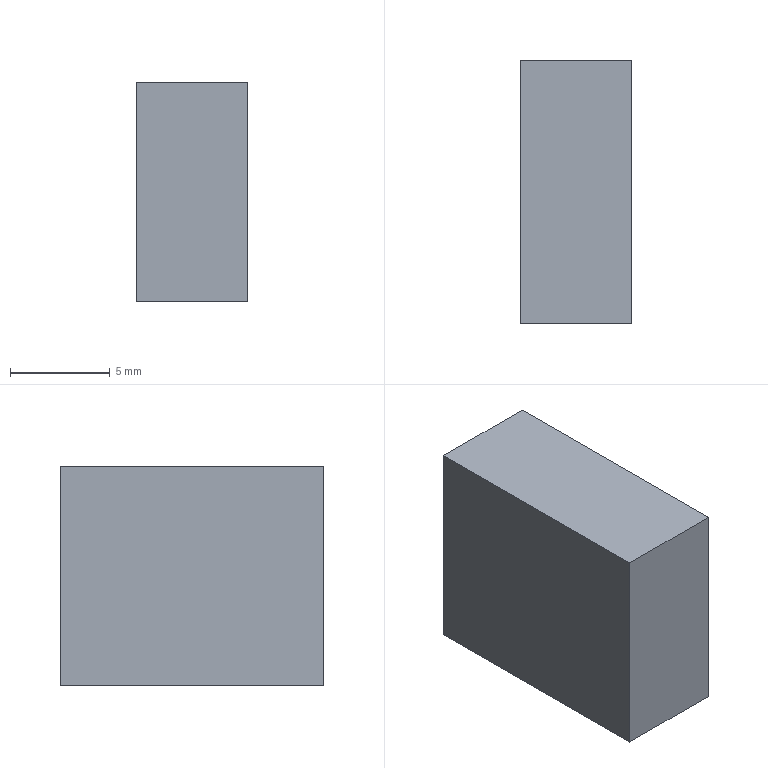CAM job | Mastercam | mm | 8 operations | part box 5.6 x 13.2 x 11
1. Facing | 24 - 100 平铣刀
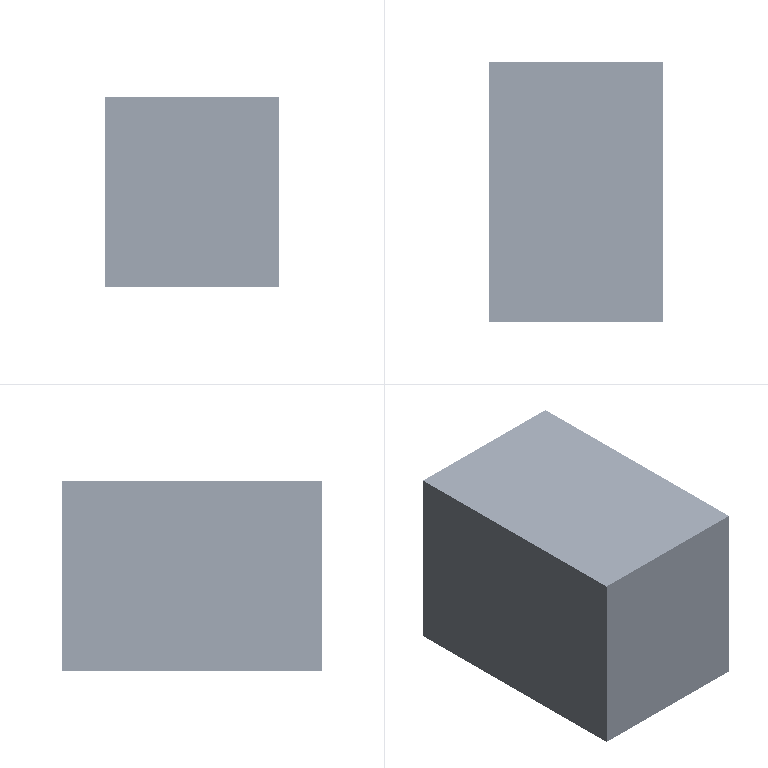2. Contour (Ramp) | 9 - 10 平铣刀
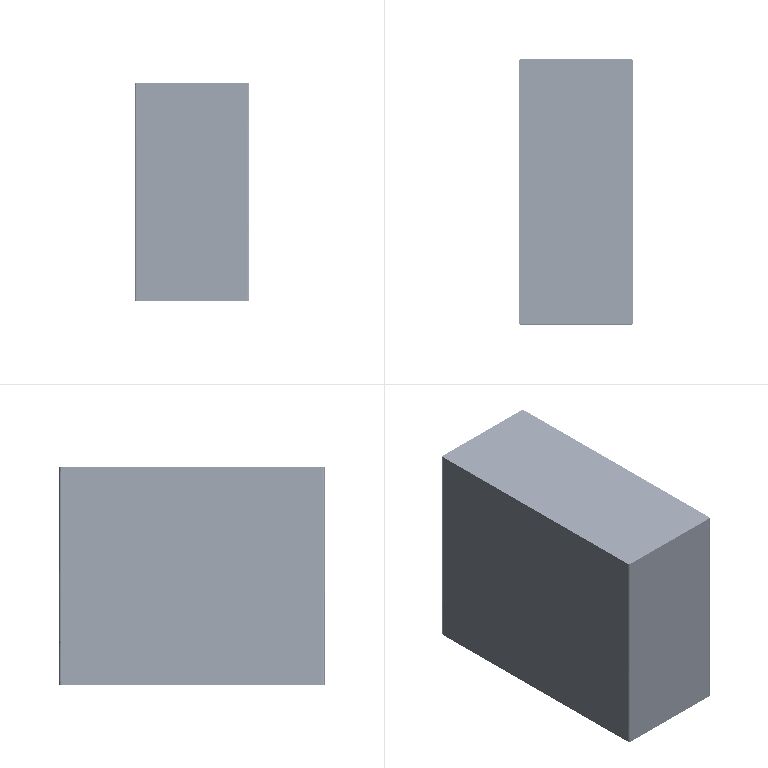3. Contour (2D) | 10 - 10 平铣刀
4. Drill/Counterbore | 5 - 4 倒角刀
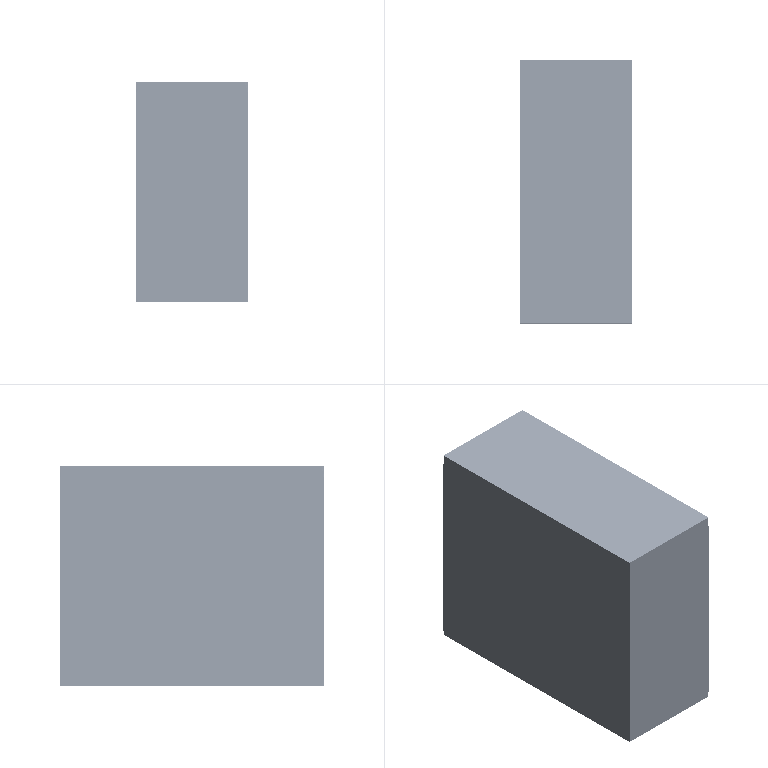5. Contour (2D chamfer) | 5 - 4 倒角刀
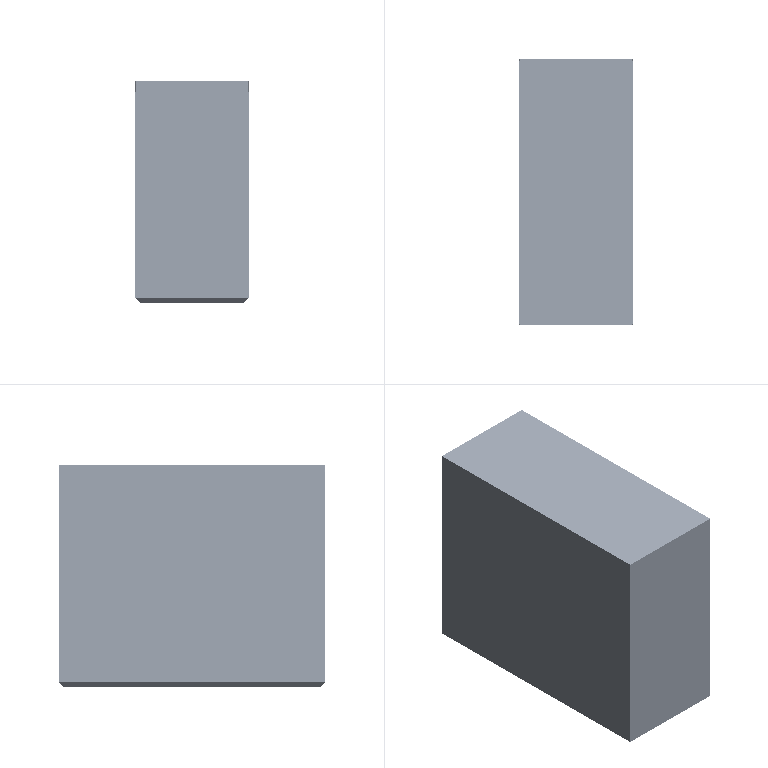6. Facing | 24 - 100 平铣刀
7. Contour (2D chamfer) | 5 - 4 倒角刀
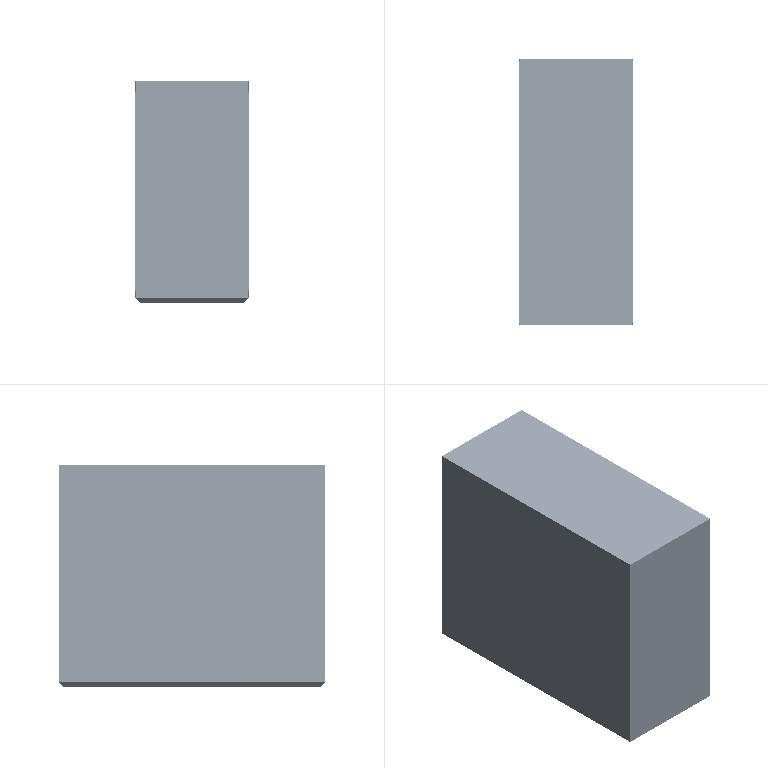8. Drill/Counterbore | 5 - 4 倒角刀